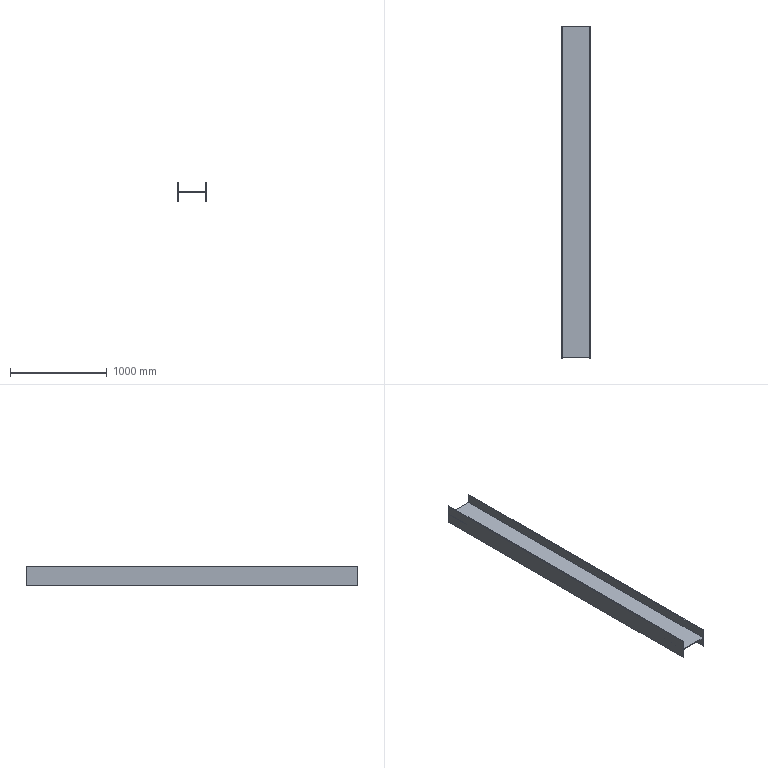Component | NX | F2 | 1 solid | 14 faces | box 300 x 3440 x 200 mm | volume 18823680 mm3 | plane 14
STEP:
#1=CARTESIAN_POINT('',(0.,0.,0.));
#2=DIRECTION('',(0.,0.,1.));
#3=DIRECTION('',(1.,0.,0.));
#4=AXIS2_PLACEMENT_3D('',#1,#2,#3);
#5=CARTESIAN_POINT('',(6772.,-266.,1440.));
#6=VERTEX_POINT('',#5);
#7=CARTESIAN_POINT('',(6772.,-266.,1536.));
#8=VERTEX_POINT('',#7);
#9=CARTESIAN_POINT('',(6772.,-266.,1440.));
#10=DIRECTION('',(0.,0.,1.));
#11=VECTOR('',#10,1.);
#12=LINE('',#9,#11);
#13=CARTESIAN_POINT('',(6772.,-3706.,1440.));
#14=DIRECTION('',(-1.,0.,0.));
#15=DIRECTION('',(0.,1.,0.));
#16=AXIS2_PLACEMENT_3D('',#13,#14,#15);
#17=PLANE('',#16);
#18=CARTESIAN_POINT('',(3440.,0.));
#19=DIRECTION('',(0.,-1.));
#20=VECTOR('',#19,1.);
#21=LINE('',#18,#20);
#22=(GEOMETRIC_REPRESENTATION_CONTEXT(2)PARAMETRIC_REPRESENTATION_CONTEXT()REPRESENTATION_CONTEXT('',''));
#23=DEFINITIONAL_REPRESENTATION('',(#21),#22);
#24=PCURVE('',#17,#23);
#25=CARTESIAN_POINT('',(6480.,-266.,1640.));
#26=DIRECTION('',(0.,-1.,0.));
#27=DIRECTION('',(-1.,0.,0.));
#28=AXIS2_PLACEMENT_3D('',#25,#26,#27);
#29=PLANE('',#28);
#30=CARTESIAN_POINT('',(-292.,200.));
#31=DIRECTION('',(0.,-1.));
#32=VECTOR('',#31,1.);
#33=LINE('',#30,#32);
#34=(GEOMETRIC_REPRESENTATION_CONTEXT(2)PARAMETRIC_REPRESENTATION_CONTEXT()REPRESENTATION_CONTEXT('',''));
#35=DEFINITIONAL_REPRESENTATION('',(#33),#34);
#36=PCURVE('',#29,#35);
#37=SURFACE_CURVE('',#12,(#24,#36),.PCURVE_S1.);
#38=EDGE_CURVE('',#6,#8,#37,.T.);
#39=ORIENTED_EDGE('',*,*,#38,.F.);
#40=CARTESIAN_POINT('',(6772.,-3706.,1440.));
#41=VERTEX_POINT('',#40);
#42=CARTESIAN_POINT('',(6772.,-3706.,1440.));
#43=DIRECTION('',(0.,1.,0.));
#44=VECTOR('',#43,1.);
#45=LINE('',#42,#44);
#46=CARTESIAN_POINT('',(0.,0.));
#47=DIRECTION('',(1.,0.));
#48=VECTOR('',#47,1.);
#49=LINE('',#46,#48);
#50=(GEOMETRIC_REPRESENTATION_CONTEXT(2)PARAMETRIC_REPRESENTATION_CONTEXT()REPRESENTATION_CONTEXT('',''));
#51=DEFINITIONAL_REPRESENTATION('',(#49),#50);
#52=PCURVE('',#17,#51);
#53=CARTESIAN_POINT('',(6780.,-3706.,1440.));
#54=DIRECTION('',(0.,0.,-1.));
#55=DIRECTION('',(0.,1.,0.));
#56=AXIS2_PLACEMENT_3D('',#53,#54,#55);
#57=PLANE('',#56);
#58=CARTESIAN_POINT('',(0.,-8.));
#59=DIRECTION('',(1.,0.));
#60=VECTOR('',#59,1.);
#61=LINE('',#58,#60);
#62=(GEOMETRIC_REPRESENTATION_CONTEXT(2)PARAMETRIC_REPRESENTATION_CONTEXT()REPRESENTATION_CONTEXT('',''));
#63=DEFINITIONAL_REPRESENTATION('',(#61),#62);
#64=PCURVE('',#57,#63);
#65=SURFACE_CURVE('',#45,(#52,#64),.PCURVE_S1.);
#66=EDGE_CURVE('',#41,#6,#65,.T.);
#67=ORIENTED_EDGE('',*,*,#66,.F.);
#68=CARTESIAN_POINT('',(6772.,-3706.,1536.));
#69=VERTEX_POINT('',#68);
#70=CARTESIAN_POINT('',(6772.,-3706.,1440.));
#71=DIRECTION('',(0.,0.,1.));
#72=VECTOR('',#71,1.);
#73=LINE('',#70,#72);
#74=CARTESIAN_POINT('',(0.,0.));
#75=DIRECTION('',(0.,-1.));
#76=VECTOR('',#75,1.);
#77=LINE('',#74,#76);
#78=(GEOMETRIC_REPRESENTATION_CONTEXT(2)PARAMETRIC_REPRESENTATION_CONTEXT()REPRESENTATION_CONTEXT('',''));
#79=DEFINITIONAL_REPRESENTATION('',(#77),#78);
#80=PCURVE('',#17,#79);
#81=CARTESIAN_POINT('',(6480.,-3706.,1640.));
#82=DIRECTION('',(0.,-1.,0.));
#83=DIRECTION('',(-1.,0.,0.));
#84=AXIS2_PLACEMENT_3D('',#81,#82,#83);
#85=PLANE('',#84);
#86=CARTESIAN_POINT('',(-292.,200.));
#87=DIRECTION('',(0.,-1.));
#88=VECTOR('',#87,1.);
#89=LINE('',#86,#88);
#90=(GEOMETRIC_REPRESENTATION_CONTEXT(2)PARAMETRIC_REPRESENTATION_CONTEXT()REPRESENTATION_CONTEXT('',''));
#91=DEFINITIONAL_REPRESENTATION('',(#89),#90);
#92=PCURVE('',#85,#91);
#93=SURFACE_CURVE('',#73,(#80,#92),.PCURVE_S1.);
#94=EDGE_CURVE('',#41,#69,#93,.T.);
#95=ORIENTED_EDGE('',*,*,#94,.T.);
#96=CARTESIAN_POINT('',(6772.,-3706.,1536.));
#97=DIRECTION('',(0.,1.,0.));
#98=VECTOR('',#97,1.);
#99=LINE('',#96,#98);
#100=CARTESIAN_POINT('',(0.,-96.));
#101=DIRECTION('',(1.,0.));
#102=VECTOR('',#101,1.);
#103=LINE('',#100,#102);
#104=(GEOMETRIC_REPRESENTATION_CONTEXT(2)PARAMETRIC_REPRESENTATION_CONTEXT()REPRESENTATION_CONTEXT('',''));
#105=DEFINITIONAL_REPRESENTATION('',(#103),#104);
#106=PCURVE('',#17,#105);
#107=CARTESIAN_POINT('',(6772.,-3706.,1536.));
#108=DIRECTION('',(0.,0.,-1.));
#109=DIRECTION('',(0.,1.,0.));
#110=AXIS2_PLACEMENT_3D('',#107,#108,#109);
#111=PLANE('',#110);
#112=CARTESIAN_POINT('',(0.,0.));
#113=DIRECTION('',(1.,0.));
#114=VECTOR('',#113,1.);
#115=LINE('',#112,#114);
#116=(GEOMETRIC_REPRESENTATION_CONTEXT(2)PARAMETRIC_REPRESENTATION_CONTEXT()REPRESENTATION_CONTEXT('',''));
#117=DEFINITIONAL_REPRESENTATION('',(#115),#116);
#118=PCURVE('',#111,#117);
#119=SURFACE_CURVE('',#99,(#106,#118),.PCURVE_S1.);
#120=EDGE_CURVE('',#69,#8,#119,.T.);
#121=ORIENTED_EDGE('',*,*,#120,.T.);
#122=EDGE_LOOP('',(#39,#67,#95,#121));
#123=FACE_BOUND('',#122,.T.);
#124=ADVANCED_FACE('',(#123),#17,.T.);
#125=CARTESIAN_POINT('',(6488.,-266.,1536.));
#126=VERTEX_POINT('',#125);
#127=CARTESIAN_POINT('',(6772.,-266.,1536.));
#128=DIRECTION('',(-1.,0.,0.));
#129=VECTOR('',#128,1.);
#130=LINE('',#127,#129);
#131=CARTESIAN_POINT('',(3440.,0.));
#132=DIRECTION('',(0.,-1.));
#133=VECTOR('',#132,1.);
#134=LINE('',#131,#133);
#135=(GEOMETRIC_REPRESENTATION_CONTEXT(2)PARAMETRIC_REPRESENTATION_CONTEXT()REPRESENTATION_CONTEXT('',''));
#136=DEFINITIONAL_REPRESENTATION('',(#134),#135);
#137=PCURVE('',#111,#136);
#138=CARTESIAN_POINT('',(-292.,104.));
#139=DIRECTION('',(1.,0.));
#140=VECTOR('',#139,1.);
#141=LINE('',#138,#140);
#142=(GEOMETRIC_REPRESENTATION_CONTEXT(2)PARAMETRIC_REPRESENTATION_CONTEXT()REPRESENTATION_CONTEXT('',''));
#143=DEFINITIONAL_REPRESENTATION('',(#141),#142);
#144=PCURVE('',#29,#143);
#145=SURFACE_CURVE('',#130,(#137,#144),.PCURVE_S1.);
#146=EDGE_CURVE('',#8,#126,#145,.T.);
#147=ORIENTED_EDGE('',*,*,#146,.F.);
#148=ORIENTED_EDGE('',*,*,#120,.F.);
#149=CARTESIAN_POINT('',(6488.,-3706.,1536.));
#150=VERTEX_POINT('',#149);
#151=CARTESIAN_POINT('',(6772.,-3706.,1536.));
#152=DIRECTION('',(-1.,0.,0.));
#153=VECTOR('',#152,1.);
#154=LINE('',#151,#153);
#155=CARTESIAN_POINT('',(0.,0.));
#156=DIRECTION('',(0.,-1.));
#157=VECTOR('',#156,1.);
#158=LINE('',#155,#157);
#159=(GEOMETRIC_REPRESENTATION_CONTEXT(2)PARAMETRIC_REPRESENTATION_CONTEXT()REPRESENTATION_CONTEXT('',''));
#160=DEFINITIONAL_REPRESENTATION('',(#158),#159);
#161=PCURVE('',#111,#160);
#162=CARTESIAN_POINT('',(-292.,104.));
#163=DIRECTION('',(1.,0.));
#164=VECTOR('',#163,1.);
#165=LINE('',#162,#164);
#166=(GEOMETRIC_REPRESENTATION_CONTEXT(2)PARAMETRIC_REPRESENTATION_CONTEXT()REPRESENTATION_CONTEXT('',''));
#167=DEFINITIONAL_REPRESENTATION('',(#165),#166);
#168=PCURVE('',#85,#167);
#169=SURFACE_CURVE('',#154,(#161,#168),.PCURVE_S1.);
#170=EDGE_CURVE('',#69,#150,#169,.T.);
#171=ORIENTED_EDGE('',*,*,#170,.T.);
#172=CARTESIAN_POINT('',(6488.,-3706.,1536.));
#173=DIRECTION('',(0.,1.,0.));
#174=VECTOR('',#173,1.);
#175=LINE('',#172,#174);
#176=CARTESIAN_POINT('',(0.,-284.));
#177=DIRECTION('',(1.,0.));
#178=VECTOR('',#177,1.);
#179=LINE('',#176,#178);
#180=(GEOMETRIC_REPRESENTATION_CONTEXT(2)PARAMETRIC_REPRESENTATION_CONTEXT()REPRESENTATION_CONTEXT('',''));
#181=DEFINITIONAL_REPRESENTATION('',(#179),#180);
#182=PCURVE('',#111,#181);
#183=CARTESIAN_POINT('',(6488.,-3706.,1536.));
#184=DIRECTION('',(1.,0.,0.));
#185=DIRECTION('',(0.,-1.,0.));
#186=AXIS2_PLACEMENT_3D('',#183,#184,#185);
#187=PLANE('',#186);
#188=CARTESIAN_POINT('',(0.,0.));
#189=DIRECTION('',(-1.,0.));
#190=VECTOR('',#189,1.);
#191=LINE('',#188,#190);
#192=(GEOMETRIC_REPRESENTATION_CONTEXT(2)PARAMETRIC_REPRESENTATION_CONTEXT()REPRESENTATION_CONTEXT('',''));
#193=DEFINITIONAL_REPRESENTATION('',(#191),#192);
#194=PCURVE('',#187,#193);
#195=SURFACE_CURVE('',#175,(#182,#194),.PCURVE_S1.);
#196=EDGE_CURVE('',#150,#126,#195,.T.);
#197=ORIENTED_EDGE('',*,*,#196,.T.);
#198=EDGE_LOOP('',(#147,#148,#171,#197));
#199=FACE_BOUND('',#198,.T.);
#200=ADVANCED_FACE('',(#199),#111,.T.);
#201=CARTESIAN_POINT('',(6488.,-266.,1440.));
#202=VERTEX_POINT('',#201);
#203=CARTESIAN_POINT('',(6488.,-266.,1536.));
#204=DIRECTION('',(0.,0.,-1.));
#205=VECTOR('',#204,1.);
#206=LINE('',#203,#205);
#207=CARTESIAN_POINT('',(-3440.,0.));
#208=DIRECTION('',(0.,1.));
#209=VECTOR('',#208,1.);
#210=LINE('',#207,#209);
#211=(GEOMETRIC_REPRESENTATION_CONTEXT(2)PARAMETRIC_REPRESENTATION_CONTEXT()REPRESENTATION_CONTEXT('',''));
#212=DEFINITIONAL_REPRESENTATION('',(#210),#211);
#213=PCURVE('',#187,#212);
#214=CARTESIAN_POINT('',(-8.,104.));
#215=DIRECTION('',(0.,1.));
#216=VECTOR('',#215,1.);
#217=LINE('',#214,#216);
#218=(GEOMETRIC_REPRESENTATION_CONTEXT(2)PARAMETRIC_REPRESENTATION_CONTEXT()REPRESENTATION_CONTEXT('',''));
#219=DEFINITIONAL_REPRESENTATION('',(#217),#218);
#220=PCURVE('',#29,#219);
#221=SURFACE_CURVE('',#206,(#213,#220),.PCURVE_S1.);
#222=EDGE_CURVE('',#126,#202,#221,.T.);
#223=ORIENTED_EDGE('',*,*,#222,.F.);
#224=ORIENTED_EDGE('',*,*,#196,.F.);
#225=CARTESIAN_POINT('',(6488.,-3706.,1440.));
#226=VERTEX_POINT('',#225);
#227=CARTESIAN_POINT('',(6488.,-3706.,1536.));
#228=DIRECTION('',(0.,0.,-1.));
#229=VECTOR('',#228,1.);
#230=LINE('',#227,#229);
#231=CARTESIAN_POINT('',(0.,0.));
#232=DIRECTION('',(0.,1.));
#233=VECTOR('',#232,1.);
#234=LINE('',#231,#233);
#235=(GEOMETRIC_REPRESENTATION_CONTEXT(2)PARAMETRIC_REPRESENTATION_CONTEXT()REPRESENTATION_CONTEXT('',''));
#236=DEFINITIONAL_REPRESENTATION('',(#234),#235);
#237=PCURVE('',#187,#236);
#238=CARTESIAN_POINT('',(-8.,104.));
#239=DIRECTION('',(0.,1.));
#240=VECTOR('',#239,1.);
#241=LINE('',#238,#240);
#242=(GEOMETRIC_REPRESENTATION_CONTEXT(2)PARAMETRIC_REPRESENTATION_CONTEXT()REPRESENTATION_CONTEXT('',''));
#243=DEFINITIONAL_REPRESENTATION('',(#241),#242);
#244=PCURVE('',#85,#243);
#245=SURFACE_CURVE('',#230,(#237,#244),.PCURVE_S1.);
#246=EDGE_CURVE('',#150,#226,#245,.T.);
#247=ORIENTED_EDGE('',*,*,#246,.T.);
#248=CARTESIAN_POINT('',(6488.,-3706.,1440.));
#249=DIRECTION('',(0.,1.,0.));
#250=VECTOR('',#249,1.);
#251=LINE('',#248,#250);
#252=CARTESIAN_POINT('',(0.,96.));
#253=DIRECTION('',(-1.,0.));
#254=VECTOR('',#253,1.);
#255=LINE('',#252,#254);
#256=(GEOMETRIC_REPRESENTATION_CONTEXT(2)PARAMETRIC_REPRESENTATION_CONTEXT()REPRESENTATION_CONTEXT('',''));
#257=DEFINITIONAL_REPRESENTATION('',(#255),#256);
#258=PCURVE('',#187,#257);
#259=CARTESIAN_POINT('',(6488.,-3706.,1440.));
#260=DIRECTION('',(0.,0.,-1.));
#261=DIRECTION('',(0.,1.,0.));
#262=AXIS2_PLACEMENT_3D('',#259,#260,#261);
#263=PLANE('',#262);
#264=CARTESIAN_POINT('',(0.,0.));
#265=DIRECTION('',(1.,0.));
#266=VECTOR('',#265,1.);
#267=LINE('',#264,#266);
#268=(GEOMETRIC_REPRESENTATION_CONTEXT(2)PARAMETRIC_REPRESENTATION_CONTEXT()REPRESENTATION_CONTEXT('',''));
#269=DEFINITIONAL_REPRESENTATION('',(#267),#268);
#270=PCURVE('',#263,#269);
#271=SURFACE_CURVE('',#251,(#258,#270),.PCURVE_S1.);
#272=EDGE_CURVE('',#226,#202,#271,.T.);
#273=ORIENTED_EDGE('',*,*,#272,.T.);
#274=EDGE_LOOP('',(#223,#224,#247,#273));
#275=FACE_BOUND('',#274,.T.);
#276=ADVANCED_FACE('',(#275),#187,.T.);
#277=CARTESIAN_POINT('',(6480.,-266.,1440.));
#278=VERTEX_POINT('',#277);
#279=CARTESIAN_POINT('',(6488.,-266.,1440.));
#280=DIRECTION('',(-1.,0.,0.));
#281=VECTOR('',#280,1.);
#282=LINE('',#279,#281);
#283=CARTESIAN_POINT('',(3440.,0.));
#284=DIRECTION('',(0.,-1.));
#285=VECTOR('',#284,1.);
#286=LINE('',#283,#285);
#287=(GEOMETRIC_REPRESENTATION_CONTEXT(2)PARAMETRIC_REPRESENTATION_CONTEXT()REPRESENTATION_CONTEXT('',''));
#288=DEFINITIONAL_REPRESENTATION('',(#286),#287);
#289=PCURVE('',#263,#288);
#290=CARTESIAN_POINT('',(-8.,200.));
#291=DIRECTION('',(1.,0.));
#292=VECTOR('',#291,1.);
#293=LINE('',#290,#292);
#294=(GEOMETRIC_REPRESENTATION_CONTEXT(2)PARAMETRIC_REPRESENTATION_CONTEXT()REPRESENTATION_CONTEXT('',''));
#295=DEFINITIONAL_REPRESENTATION('',(#293),#294);
#296=PCURVE('',#29,#295);
#297=SURFACE_CURVE('',#282,(#289,#296),.PCURVE_S1.);
#298=EDGE_CURVE('',#202,#278,#297,.T.);
#299=ORIENTED_EDGE('',*,*,#298,.F.);
#300=ORIENTED_EDGE('',*,*,#272,.F.);
#301=CARTESIAN_POINT('',(6480.,-3706.,1440.));
#302=VERTEX_POINT('',#301);
#303=CARTESIAN_POINT('',(6488.,-3706.,1440.));
#304=DIRECTION('',(-1.,0.,0.));
#305=VECTOR('',#304,1.);
#306=LINE('',#303,#305);
#307=CARTESIAN_POINT('',(0.,0.));
#308=DIRECTION('',(0.,-1.));
#309=VECTOR('',#308,1.);
#310=LINE('',#307,#309);
#311=(GEOMETRIC_REPRESENTATION_CONTEXT(2)PARAMETRIC_REPRESENTATION_CONTEXT()REPRESENTATION_CONTEXT('',''));
#312=DEFINITIONAL_REPRESENTATION('',(#310),#311);
#313=PCURVE('',#263,#312);
#314=CARTESIAN_POINT('',(-8.,200.));
#315=DIRECTION('',(1.,0.));
#316=VECTOR('',#315,1.);
#317=LINE('',#314,#316);
#318=(GEOMETRIC_REPRESENTATION_CONTEXT(2)PARAMETRIC_REPRESENTATION_CONTEXT()REPRESENTATION_CONTEXT('',''));
#319=DEFINITIONAL_REPRESENTATION('',(#317),#318);
#320=PCURVE('',#85,#319);
#321=SURFACE_CURVE('',#306,(#313,#320),.PCURVE_S1.);
#322=EDGE_CURVE('',#226,#302,#321,.T.);
#323=ORIENTED_EDGE('',*,*,#322,.T.);
#324=CARTESIAN_POINT('',(6480.,-3706.,1440.));
#325=DIRECTION('',(0.,1.,0.));
#326=VECTOR('',#325,1.);
#327=LINE('',#324,#326);
#328=CARTESIAN_POINT('',(0.,-8.));
#329=DIRECTION('',(1.,0.));
#330=VECTOR('',#329,1.);
#331=LINE('',#328,#330);
#332=(GEOMETRIC_REPRESENTATION_CONTEXT(2)PARAMETRIC_REPRESENTATION_CONTEXT()REPRESENTATION_CONTEXT('',''));
#333=DEFINITIONAL_REPRESENTATION('',(#331),#332);
#334=PCURVE('',#263,#333);
#335=CARTESIAN_POINT('',(6480.,-3706.,1440.));
#336=DIRECTION('',(-1.,0.,0.));
#337=DIRECTION('',(0.,1.,0.));
#338=AXIS2_PLACEMENT_3D('',#335,#336,#337);
#339=PLANE('',#338);
#340=CARTESIAN_POINT('',(0.,0.));
#341=DIRECTION('',(1.,0.));
#342=VECTOR('',#341,1.);
#343=LINE('',#340,#342);
#344=(GEOMETRIC_REPRESENTATION_CONTEXT(2)PARAMETRIC_REPRESENTATION_CONTEXT()REPRESENTATION_CONTEXT('',''));
#345=DEFINITIONAL_REPRESENTATION('',(#343),#344);
#346=PCURVE('',#339,#345);
#347=SURFACE_CURVE('',#327,(#334,#346),.PCURVE_S1.);
#348=EDGE_CURVE('',#302,#278,#347,.T.);
#349=ORIENTED_EDGE('',*,*,#348,.T.);
#350=EDGE_LOOP('',(#299,#300,#323,#349));
#351=FACE_BOUND('',#350,.T.);
#352=ADVANCED_FACE('',(#351),#263,.T.);
#353=CARTESIAN_POINT('',(6480.,-266.,1640.));
#354=VERTEX_POINT('',#353);
#355=CARTESIAN_POINT('',(6480.,-266.,1440.));
#356=DIRECTION('',(0.,0.,1.));
#357=VECTOR('',#356,1.);
#358=LINE('',#355,#357);
#359=CARTESIAN_POINT('',(3440.,0.));
#360=DIRECTION('',(0.,-1.));
#361=VECTOR('',#360,1.);
#362=LINE('',#359,#361);
#363=(GEOMETRIC_REPRESENTATION_CONTEXT(2)PARAMETRIC_REPRESENTATION_CONTEXT()REPRESENTATION_CONTEXT('',''));
#364=DEFINITIONAL_REPRESENTATION('',(#362),#363);
#365=PCURVE('',#339,#364);
#366=CARTESIAN_POINT('',(0.,200.));
#367=DIRECTION('',(0.,-1.));
#368=VECTOR('',#367,1.);
#369=LINE('',#366,#368);
#370=(GEOMETRIC_REPRESENTATION_CONTEXT(2)PARAMETRIC_REPRESENTATION_CONTEXT()REPRESENTATION_CONTEXT('',''));
#371=DEFINITIONAL_REPRESENTATION('',(#369),#370);
#372=PCURVE('',#29,#371);
#373=SURFACE_CURVE('',#358,(#365,#372),.PCURVE_S1.);
#374=EDGE_CURVE('',#278,#354,#373,.T.);
#375=ORIENTED_EDGE('',*,*,#374,.F.);
#376=ORIENTED_EDGE('',*,*,#348,.F.);
#377=CARTESIAN_POINT('',(6480.,-3706.,1640.));
#378=VERTEX_POINT('',#377);
#379=CARTESIAN_POINT('',(6480.,-3706.,1440.));
#380=DIRECTION('',(0.,0.,1.));
#381=VECTOR('',#380,1.);
#382=LINE('',#379,#381);
#383=CARTESIAN_POINT('',(0.,0.));
#384=DIRECTION('',(0.,-1.));
#385=VECTOR('',#384,1.);
#386=LINE('',#383,#385);
#387=(GEOMETRIC_REPRESENTATION_CONTEXT(2)PARAMETRIC_REPRESENTATION_CONTEXT()REPRESENTATION_CONTEXT('',''));
#388=DEFINITIONAL_REPRESENTATION('',(#386),#387);
#389=PCURVE('',#339,#388);
#390=CARTESIAN_POINT('',(0.,200.));
#391=DIRECTION('',(0.,-1.));
#392=VECTOR('',#391,1.);
#393=LINE('',#390,#392);
#394=(GEOMETRIC_REPRESENTATION_CONTEXT(2)PARAMETRIC_REPRESENTATION_CONTEXT()REPRESENTATION_CONTEXT('',''));
#395=DEFINITIONAL_REPRESENTATION('',(#393),#394);
#396=PCURVE('',#85,#395);
#397=SURFACE_CURVE('',#382,(#389,#396),.PCURVE_S1.);
#398=EDGE_CURVE('',#302,#378,#397,.T.);
#399=ORIENTED_EDGE('',*,*,#398,.T.);
#400=CARTESIAN_POINT('',(6480.,-3706.,1640.));
#401=DIRECTION('',(0.,1.,0.));
#402=VECTOR('',#401,1.);
#403=LINE('',#400,#402);
#404=CARTESIAN_POINT('',(0.,-200.));
#405=DIRECTION('',(1.,0.));
#406=VECTOR('',#405,1.);
#407=LINE('',#404,#406);
#408=(GEOMETRIC_REPRESENTATION_CONTEXT(2)PARAMETRIC_REPRESENTATION_CONTEXT()REPRESENTATION_CONTEXT('',''));
#409=DEFINITIONAL_REPRESENTATION('',(#407),#408);
#410=PCURVE('',#339,#409);
#411=CARTESIAN_POINT('',(6480.,-3706.,1640.));
#412=DIRECTION('',(0.,0.,1.));
#413=DIRECTION('',(0.,-1.,0.));
#414=AXIS2_PLACEMENT_3D('',#411,#412,#413);
#415=PLANE('',#414);
#416=CARTESIAN_POINT('',(0.,0.));
#417=DIRECTION('',(-1.,0.));
#418=VECTOR('',#417,1.);
#419=LINE('',#416,#418);
#420=(GEOMETRIC_REPRESENTATION_CONTEXT(2)PARAMETRIC_REPRESENTATION_CONTEXT()REPRESENTATION_CONTEXT('',''));
#421=DEFINITIONAL_REPRESENTATION('',(#419),#420);
#422=PCURVE('',#415,#421);
#423=SURFACE_CURVE('',#403,(#410,#422),.PCURVE_S1.);
#424=EDGE_CURVE('',#378,#354,#423,.T.);
#425=ORIENTED_EDGE('',*,*,#424,.T.);
#426=EDGE_LOOP('',(#375,#376,#399,#425));
#427=FACE_BOUND('',#426,.T.);
#428=ADVANCED_FACE('',(#427),#339,.T.);
#429=CARTESIAN_POINT('',(6488.,-266.,1640.));
#430=VERTEX_POINT('',#429);
#431=CARTESIAN_POINT('',(6480.,-266.,1640.));
#432=DIRECTION('',(1.,0.,0.));
#433=VECTOR('',#432,1.);
#434=LINE('',#431,#433);
#435=CARTESIAN_POINT('',(-3440.,0.));
#436=DIRECTION('',(0.,1.));
#437=VECTOR('',#436,1.);
#438=LINE('',#435,#437);
#439=(GEOMETRIC_REPRESENTATION_CONTEXT(2)PARAMETRIC_REPRESENTATION_CONTEXT()REPRESENTATION_CONTEXT('',''));
#440=DEFINITIONAL_REPRESENTATION('',(#438),#439);
#441=PCURVE('',#415,#440);
#442=CARTESIAN_POINT('',(0.,0.));
#443=DIRECTION('',(-1.,0.));
#444=VECTOR('',#443,1.);
#445=LINE('',#442,#444);
#446=(GEOMETRIC_REPRESENTATION_CONTEXT(2)PARAMETRIC_REPRESENTATION_CONTEXT()REPRESENTATION_CONTEXT('',''));
#447=DEFINITIONAL_REPRESENTATION('',(#445),#446);
#448=PCURVE('',#29,#447);
#449=SURFACE_CURVE('',#434,(#441,#448),.PCURVE_S1.);
#450=EDGE_CURVE('',#354,#430,#449,.T.);
#451=ORIENTED_EDGE('',*,*,#450,.F.);
#452=ORIENTED_EDGE('',*,*,#424,.F.);
#453=CARTESIAN_POINT('',(6488.,-3706.,1640.));
#454=VERTEX_POINT('',#453);
#455=CARTESIAN_POINT('',(6480.,-3706.,1640.));
#456=DIRECTION('',(1.,0.,0.));
#457=VECTOR('',#456,1.);
#458=LINE('',#455,#457);
#459=CARTESIAN_POINT('',(0.,0.));
#460=DIRECTION('',(0.,1.));
#461=VECTOR('',#460,1.);
#462=LINE('',#459,#461);
#463=(GEOMETRIC_REPRESENTATION_CONTEXT(2)PARAMETRIC_REPRESENTATION_CONTEXT()REPRESENTATION_CONTEXT('',''));
#464=DEFINITIONAL_REPRESENTATION('',(#462),#463);
#465=PCURVE('',#415,#464);
#466=CARTESIAN_POINT('',(0.,0.));
#467=DIRECTION('',(-1.,0.));
#468=VECTOR('',#467,1.);
#469=LINE('',#466,#468);
#470=(GEOMETRIC_REPRESENTATION_CONTEXT(2)PARAMETRIC_REPRESENTATION_CONTEXT()REPRESENTATION_CONTEXT('',''));
#471=DEFINITIONAL_REPRESENTATION('',(#469),#470);
#472=PCURVE('',#85,#471);
#473=SURFACE_CURVE('',#458,(#465,#472),.PCURVE_S1.);
#474=EDGE_CURVE('',#378,#454,#473,.T.);
#475=ORIENTED_EDGE('',*,*,#474,.T.);
#476=CARTESIAN_POINT('',(6488.,-3706.,1640.));
#477=DIRECTION('',(0.,1.,0.));
#478=VECTOR('',#477,1.);
#479=LINE('',#476,#478);
#480=CARTESIAN_POINT('',(0.,8.));
#481=DIRECTION('',(-1.,0.));
#482=VECTOR('',#481,1.);
#483=LINE('',#480,#482);
#484=(GEOMETRIC_REPRESENTATION_CONTEXT(2)PARAMETRIC_REPRESENTATION_CONTEXT()REPRESENTATION_CONTEXT('',''));
#485=DEFINITIONAL_REPRESENTATION('',(#483),#484);
#486=PCURVE('',#415,#485);
#487=CARTESIAN_POINT('',(6488.,-3706.,1640.));
#488=DIRECTION('',(1.,0.,0.));
#489=DIRECTION('',(0.,-1.,0.));
#490=AXIS2_PLACEMENT_3D('',#487,#488,#489);
#491=PLANE('',#490);
#492=CARTESIAN_POINT('',(0.,0.));
#493=DIRECTION('',(-1.,0.));
#494=VECTOR('',#493,1.);
#495=LINE('',#492,#494);
#496=(GEOMETRIC_REPRESENTATION_CONTEXT(2)PARAMETRIC_REPRESENTATION_CONTEXT()REPRESENTATION_CONTEXT('',''));
#497=DEFINITIONAL_REPRESENTATION('',(#495),#496);
#498=PCURVE('',#491,#497);
#499=SURFACE_CURVE('',#479,(#486,#498),.PCURVE_S1.);
#500=EDGE_CURVE('',#454,#430,#499,.T.);
#501=ORIENTED_EDGE('',*,*,#500,.T.);
#502=EDGE_LOOP('',(#451,#452,#475,#501));
#503=FACE_BOUND('',#502,.T.);
#504=ADVANCED_FACE('',(#503),#415,.T.);
#505=CARTESIAN_POINT('',(6488.,-266.,1544.));
#506=VERTEX_POINT('',#505);
#507=CARTESIAN_POINT('',(6488.,-266.,1640.));
#508=DIRECTION('',(0.,0.,-1.));
#509=VECTOR('',#508,1.);
#510=LINE('',#507,#509);
#511=CARTESIAN_POINT('',(-3440.,0.));
#512=DIRECTION('',(0.,1.));
#513=VECTOR('',#512,1.);
#514=LINE('',#511,#513);
#515=(GEOMETRIC_REPRESENTATION_CONTEXT(2)PARAMETRIC_REPRESENTATION_CONTEXT()REPRESENTATION_CONTEXT('',''));
#516=DEFINITIONAL_REPRESENTATION('',(#514),#515);
#517=PCURVE('',#491,#516);
#518=CARTESIAN_POINT('',(-8.,0.));
#519=DIRECTION('',(0.,1.));
#520=VECTOR('',#519,1.);
#521=LINE('',#518,#520);
#522=(GEOMETRIC_REPRESENTATION_CONTEXT(2)PARAMETRIC_REPRESENTATION_CONTEXT()REPRESENTATION_CONTEXT('',''));
#523=DEFINITIONAL_REPRESENTATION('',(#521),#522);
#524=PCURVE('',#29,#523);
#525=SURFACE_CURVE('',#510,(#517,#524),.PCURVE_S1.);
#526=EDGE_CURVE('',#430,#506,#525,.T.);
#527=ORIENTED_EDGE('',*,*,#526,.F.);
#528=ORIENTED_EDGE('',*,*,#500,.F.);
#529=CARTESIAN_POINT('',(6488.,-3706.,1544.));
#530=VERTEX_POINT('',#529);
#531=CARTESIAN_POINT('',(6488.,-3706.,1640.));
#532=DIRECTION('',(0.,0.,-1.));
#533=VECTOR('',#532,1.);
#534=LINE('',#531,#533);
#535=CARTESIAN_POINT('',(0.,0.));
#536=DIRECTION('',(0.,1.));
#537=VECTOR('',#536,1.);
#538=LINE('',#535,#537);
#539=(GEOMETRIC_REPRESENTATION_CONTEXT(2)PARAMETRIC_REPRESENTATION_CONTEXT()REPRESENTATION_CONTEXT('',''));
#540=DEFINITIONAL_REPRESENTATION('',(#538),#539);
#541=PCURVE('',#491,#540);
#542=CARTESIAN_POINT('',(-8.,0.));
#543=DIRECTION('',(0.,1.));
#544=VECTOR('',#543,1.);
#545=LINE('',#542,#544);
#546=(GEOMETRIC_REPRESENTATION_CONTEXT(2)PARAMETRIC_REPRESENTATION_CONTEXT()REPRESENTATION_CONTEXT('',''));
#547=DEFINITIONAL_REPRESENTATION('',(#545),#546);
#548=PCURVE('',#85,#547);
#549=SURFACE_CURVE('',#534,(#541,#548),.PCURVE_S1.);
#550=EDGE_CURVE('',#454,#530,#549,.T.);
#551=ORIENTED_EDGE('',*,*,#550,.T.);
#552=CARTESIAN_POINT('',(6488.,-3706.,1544.));
#553=DIRECTION('',(0.,1.,0.));
#554=VECTOR('',#553,1.);
#555=LINE('',#552,#554);
#556=CARTESIAN_POINT('',(0.,96.));
#557=DIRECTION('',(-1.,0.));
#558=VECTOR('',#557,1.);
#559=LINE('',#556,#558);
#560=(GEOMETRIC_REPRESENTATION_CONTEXT(2)PARAMETRIC_REPRESENTATION_CONTEXT()REPRESENTATION_CONTEXT('',''));
#561=DEFINITIONAL_REPRESENTATION('',(#559),#560);
#562=PCURVE('',#491,#561);
#563=CARTESIAN_POINT('',(6488.,-3706.,1544.));
#564=DIRECTION('',(0.,0.,1.));
#565=DIRECTION('',(0.,-1.,0.));
#566=AXIS2_PLACEMENT_3D('',#563,#564,#565);
#567=PLANE('',#566);
#568=CARTESIAN_POINT('',(0.,0.));
#569=DIRECTION('',(-1.,0.));
#570=VECTOR('',#569,1.);
#571=LINE('',#568,#570);
#572=(GEOMETRIC_REPRESENTATION_CONTEXT(2)PARAMETRIC_REPRESENTATION_CONTEXT()REPRESENTATION_CONTEXT('',''));
#573=DEFINITIONAL_REPRESENTATION('',(#571),#572);
#574=PCURVE('',#567,#573);
#575=SURFACE_CURVE('',#555,(#562,#574),.PCURVE_S1.);
#576=EDGE_CURVE('',#530,#506,#575,.T.);
#577=ORIENTED_EDGE('',*,*,#576,.T.);
#578=EDGE_LOOP('',(#527,#528,#551,#577));
#579=FACE_BOUND('',#578,.T.);
#580=ADVANCED_FACE('',(#579),#491,.T.);
#581=CARTESIAN_POINT('',(6772.,-266.,1544.));
#582=VERTEX_POINT('',#581);
#583=CARTESIAN_POINT('',(6488.,-266.,1544.));
#584=DIRECTION('',(1.,0.,0.));
#585=VECTOR('',#584,1.);
#586=LINE('',#583,#585);
#587=CARTESIAN_POINT('',(-3440.,0.));
#588=DIRECTION('',(0.,1.));
#589=VECTOR('',#588,1.);
#590=LINE('',#587,#589);
#591=(GEOMETRIC_REPRESENTATION_CONTEXT(2)PARAMETRIC_REPRESENTATION_CONTEXT()REPRESENTATION_CONTEXT('',''));
#592=DEFINITIONAL_REPRESENTATION('',(#590),#591);
#593=PCURVE('',#567,#592);
#594=CARTESIAN_POINT('',(-8.,96.));
#595=DIRECTION('',(-1.,0.));
#596=VECTOR('',#595,1.);
#597=LINE('',#594,#596);
#598=(GEOMETRIC_REPRESENTATION_CONTEXT(2)PARAMETRIC_REPRESENTATION_CONTEXT()REPRESENTATION_CONTEXT('',''));
#599=DEFINITIONAL_REPRESENTATION('',(#597),#598);
#600=PCURVE('',#29,#599);
#601=SURFACE_CURVE('',#586,(#593,#600),.PCURVE_S1.);
#602=EDGE_CURVE('',#506,#582,#601,.T.);
#603=ORIENTED_EDGE('',*,*,#602,.F.);
#604=ORIENTED_EDGE('',*,*,#576,.F.);
#605=CARTESIAN_POINT('',(6772.,-3706.,1544.));
#606=VERTEX_POINT('',#605);
#607=CARTESIAN_POINT('',(6488.,-3706.,1544.));
#608=DIRECTION('',(1.,0.,0.));
#609=VECTOR('',#608,1.);
#610=LINE('',#607,#609);
#611=CARTESIAN_POINT('',(0.,0.));
#612=DIRECTION('',(0.,1.));
#613=VECTOR('',#612,1.);
#614=LINE('',#611,#613);
#615=(GEOMETRIC_REPRESENTATION_CONTEXT(2)PARAMETRIC_REPRESENTATION_CONTEXT()REPRESENTATION_CONTEXT('',''));
#616=DEFINITIONAL_REPRESENTATION('',(#614),#615);
#617=PCURVE('',#567,#616);
#618=CARTESIAN_POINT('',(-8.,96.));
#619=DIRECTION('',(-1.,0.));
#620=VECTOR('',#619,1.);
#621=LINE('',#618,#620);
#622=(GEOMETRIC_REPRESENTATION_CONTEXT(2)PARAMETRIC_REPRESENTATION_CONTEXT()REPRESENTATION_CONTEXT('',''));
#623=DEFINITIONAL_REPRESENTATION('',(#621),#622);
#624=PCURVE('',#85,#623);
#625=SURFACE_CURVE('',#610,(#617,#624),.PCURVE_S1.);
#626=EDGE_CURVE('',#530,#606,#625,.T.);
#627=ORIENTED_EDGE('',*,*,#626,.T.);
#628=CARTESIAN_POINT('',(6772.,-3706.,1544.));
#629=DIRECTION('',(0.,1.,0.));
#630=VECTOR('',#629,1.);
#631=LINE('',#628,#630);
#632=CARTESIAN_POINT('',(0.,284.));
#633=DIRECTION('',(-1.,0.));
#634=VECTOR('',#633,1.);
#635=LINE('',#632,#634);
#636=(GEOMETRIC_REPRESENTATION_CONTEXT(2)PARAMETRIC_REPRESENTATION_CONTEXT()REPRESENTATION_CONTEXT('',''));
#637=DEFINITIONAL_REPRESENTATION('',(#635),#636);
#638=PCURVE('',#567,#637);
#639=CARTESIAN_POINT('',(6772.,-3706.,1544.));
#640=DIRECTION('',(-1.,0.,0.));
#641=DIRECTION('',(0.,1.,0.));
#642=AXIS2_PLACEMENT_3D('',#639,#640,#641);
#643=PLANE('',#642);
#644=CARTESIAN_POINT('',(0.,0.));
#645=DIRECTION('',(1.,0.));
#646=VECTOR('',#645,1.);
#647=LINE('',#644,#646);
#648=(GEOMETRIC_REPRESENTATION_CONTEXT(2)PARAMETRIC_REPRESENTATION_CONTEXT()REPRESENTATION_CONTEXT('',''));
#649=DEFINITIONAL_REPRESENTATION('',(#647),#648);
#650=PCURVE('',#643,#649);
#651=SURFACE_CURVE('',#631,(#638,#650),.PCURVE_S1.);
#652=EDGE_CURVE('',#606,#582,#651,.T.);
#653=ORIENTED_EDGE('',*,*,#652,.T.);
#654=EDGE_LOOP('',(#603,#604,#627,#653));
#655=FACE_BOUND('',#654,.T.);
#656=ADVANCED_FACE('',(#655),#567,.T.);
#657=CARTESIAN_POINT('',(6772.,-266.,1640.));
#658=VERTEX_POINT('',#657);
#659=CARTESIAN_POINT('',(6772.,-266.,1544.));
#660=DIRECTION('',(0.,0.,1.));
#661=VECTOR('',#660,1.);
#662=LINE('',#659,#661);
#663=CARTESIAN_POINT('',(3440.,0.));
#664=DIRECTION('',(0.,-1.));
#665=VECTOR('',#664,1.);
#666=LINE('',#663,#665);
#667=(GEOMETRIC_REPRESENTATION_CONTEXT(2)PARAMETRIC_REPRESENTATION_CONTEXT()REPRESENTATION_CONTEXT('',''));
#668=DEFINITIONAL_REPRESENTATION('',(#666),#667);
#669=PCURVE('',#643,#668);
#670=CARTESIAN_POINT('',(-292.,96.));
#671=DIRECTION('',(0.,-1.));
#672=VECTOR('',#671,1.);
#673=LINE('',#670,#672);
#674=(GEOMETRIC_REPRESENTATION_CONTEXT(2)PARAMETRIC_REPRESENTATION_CONTEXT()REPRESENTATION_CONTEXT('',''));
#675=DEFINITIONAL_REPRESENTATION('',(#673),#674);
#676=PCURVE('',#29,#675);
#677=SURFACE_CURVE('',#662,(#669,#676),.PCURVE_S1.);
#678=EDGE_CURVE('',#582,#658,#677,.T.);
#679=ORIENTED_EDGE('',*,*,#678,.F.);
#680=ORIENTED_EDGE('',*,*,#652,.F.);
#681=CARTESIAN_POINT('',(6772.,-3706.,1640.));
#682=VERTEX_POINT('',#681);
#683=CARTESIAN_POINT('',(6772.,-3706.,1544.));
#684=DIRECTION('',(0.,0.,1.));
#685=VECTOR('',#684,1.);
#686=LINE('',#683,#685);
#687=CARTESIAN_POINT('',(0.,0.));
#688=DIRECTION('',(0.,-1.));
#689=VECTOR('',#688,1.);
#690=LINE('',#687,#689);
#691=(GEOMETRIC_REPRESENTATION_CONTEXT(2)PARAMETRIC_REPRESENTATION_CONTEXT()REPRESENTATION_CONTEXT('',''));
#692=DEFINITIONAL_REPRESENTATION('',(#690),#691);
#693=PCURVE('',#643,#692);
#694=CARTESIAN_POINT('',(-292.,96.));
#695=DIRECTION('',(0.,-1.));
#696=VECTOR('',#695,1.);
#697=LINE('',#694,#696);
#698=(GEOMETRIC_REPRESENTATION_CONTEXT(2)PARAMETRIC_REPRESENTATION_CONTEXT()REPRESENTATION_CONTEXT('',''));
#699=DEFINITIONAL_REPRESENTATION('',(#697),#698);
#700=PCURVE('',#85,#699);
#701=SURFACE_CURVE('',#686,(#693,#700),.PCURVE_S1.);
#702=EDGE_CURVE('',#606,#682,#701,.T.);
#703=ORIENTED_EDGE('',*,*,#702,.T.);
#704=CARTESIAN_POINT('',(6772.,-3706.,1640.));
#705=DIRECTION('',(0.,1.,0.));
#706=VECTOR('',#705,1.);
#707=LINE('',#704,#706);
#708=CARTESIAN_POINT('',(0.,-96.));
#709=DIRECTION('',(1.,0.));
#710=VECTOR('',#709,1.);
#711=LINE('',#708,#710);
#712=(GEOMETRIC_REPRESENTATION_CONTEXT(2)PARAMETRIC_REPRESENTATION_CONTEXT()REPRESENTATION_CONTEXT('',''));
#713=DEFINITIONAL_REPRESENTATION('',(#711),#712);
#714=PCURVE('',#643,#713);
#715=CARTESIAN_POINT('',(6772.,-3706.,1640.));
#716=DIRECTION('',(0.,0.,1.));
#717=DIRECTION('',(0.,-1.,0.));
#718=AXIS2_PLACEMENT_3D('',#715,#716,#717);
#719=PLANE('',#718);
#720=CARTESIAN_POINT('',(0.,0.));
#721=DIRECTION('',(-1.,0.));
#722=VECTOR('',#721,1.);
#723=LINE('',#720,#722);
#724=(GEOMETRIC_REPRESENTATION_CONTEXT(2)PARAMETRIC_REPRESENTATION_CONTEXT()REPRESENTATION_CONTEXT('',''));
#725=DEFINITIONAL_REPRESENTATION('',(#723),#724);
#726=PCURVE('',#719,#725);
#727=SURFACE_CURVE('',#707,(#714,#726),.PCURVE_S1.);
#728=EDGE_CURVE('',#682,#658,#727,.T.);
#729=ORIENTED_EDGE('',*,*,#728,.T.);
#730=EDGE_LOOP('',(#679,#680,#703,#729));
#731=FACE_BOUND('',#730,.T.);
#732=ADVANCED_FACE('',(#731),#643,.T.);
#733=CARTESIAN_POINT('',(6780.,-266.,1640.));
#734=VERTEX_POINT('',#733);
#735=CARTESIAN_POINT('',(6772.,-266.,1640.));
#736=DIRECTION('',(1.,0.,0.));
#737=VECTOR('',#736,1.);
#738=LINE('',#735,#737);
#739=CARTESIAN_POINT('',(-3440.,0.));
#740=DIRECTION('',(0.,1.));
#741=VECTOR('',#740,1.);
#742=LINE('',#739,#741);
#743=(GEOMETRIC_REPRESENTATION_CONTEXT(2)PARAMETRIC_REPRESENTATION_CONTEXT()REPRESENTATION_CONTEXT('',''));
#744=DEFINITIONAL_REPRESENTATION('',(#742),#743);
#745=PCURVE('',#719,#744);
#746=CARTESIAN_POINT('',(-292.,0.));
#747=DIRECTION('',(-1.,0.));
#748=VECTOR('',#747,1.);
#749=LINE('',#746,#748);
#750=(GEOMETRIC_REPRESENTATION_CONTEXT(2)PARAMETRIC_REPRESENTATION_CONTEXT()REPRESENTATION_CONTEXT('',''));
#751=DEFINITIONAL_REPRESENTATION('',(#749),#750);
#752=PCURVE('',#29,#751);
#753=SURFACE_CURVE('',#738,(#745,#752),.PCURVE_S1.);
#754=EDGE_CURVE('',#658,#734,#753,.T.);
#755=ORIENTED_EDGE('',*,*,#754,.F.);
#756=ORIENTED_EDGE('',*,*,#728,.F.);
#757=CARTESIAN_POINT('',(6780.,-3706.,1640.));
#758=VERTEX_POINT('',#757);
#759=CARTESIAN_POINT('',(6772.,-3706.,1640.));
#760=DIRECTION('',(1.,0.,0.));
#761=VECTOR('',#760,1.);
#762=LINE('',#759,#761);
#763=CARTESIAN_POINT('',(0.,0.));
#764=DIRECTION('',(0.,1.));
#765=VECTOR('',#764,1.);
#766=LINE('',#763,#765);
#767=(GEOMETRIC_REPRESENTATION_CONTEXT(2)PARAMETRIC_REPRESENTATION_CONTEXT()REPRESENTATION_CONTEXT('',''));
#768=DEFINITIONAL_REPRESENTATION('',(#766),#767);
#769=PCURVE('',#719,#768);
#770=CARTESIAN_POINT('',(-292.,0.));
#771=DIRECTION('',(-1.,0.));
#772=VECTOR('',#771,1.);
#773=LINE('',#770,#772);
#774=(GEOMETRIC_REPRESENTATION_CONTEXT(2)PARAMETRIC_REPRESENTATION_CONTEXT()REPRESENTATION_CONTEXT('',''));
#775=DEFINITIONAL_REPRESENTATION('',(#773),#774);
#776=PCURVE('',#85,#775);
#777=SURFACE_CURVE('',#762,(#769,#776),.PCURVE_S1.);
#778=EDGE_CURVE('',#682,#758,#777,.T.);
#779=ORIENTED_EDGE('',*,*,#778,.T.);
#780=CARTESIAN_POINT('',(6780.,-3706.,1640.));
#781=DIRECTION('',(0.,1.,0.));
#782=VECTOR('',#781,1.);
#783=LINE('',#780,#782);
#784=CARTESIAN_POINT('',(0.,8.));
#785=DIRECTION('',(-1.,0.));
#786=VECTOR('',#785,1.);
#787=LINE('',#784,#786);
#788=(GEOMETRIC_REPRESENTATION_CONTEXT(2)PARAMETRIC_REPRESENTATION_CONTEXT()REPRESENTATION_CONTEXT('',''));
#789=DEFINITIONAL_REPRESENTATION('',(#787),#788);
#790=PCURVE('',#719,#789);
#791=CARTESIAN_POINT('',(6780.,-3706.,1640.));
#792=DIRECTION('',(1.,0.,0.));
#793=DIRECTION('',(0.,-1.,0.));
#794=AXIS2_PLACEMENT_3D('',#791,#792,#793);
#795=PLANE('',#794);
#796=CARTESIAN_POINT('',(0.,0.));
#797=DIRECTION('',(-1.,0.));
#798=VECTOR('',#797,1.);
#799=LINE('',#796,#798);
#800=(GEOMETRIC_REPRESENTATION_CONTEXT(2)PARAMETRIC_REPRESENTATION_CONTEXT()REPRESENTATION_CONTEXT('',''));
#801=DEFINITIONAL_REPRESENTATION('',(#799),#800);
#802=PCURVE('',#795,#801);
#803=SURFACE_CURVE('',#783,(#790,#802),.PCURVE_S1.);
#804=EDGE_CURVE('',#758,#734,#803,.T.);
#805=ORIENTED_EDGE('',*,*,#804,.T.);
#806=EDGE_LOOP('',(#755,#756,#779,#805));
#807=FACE_BOUND('',#806,.T.);
#808=ADVANCED_FACE('',(#807),#719,.T.);
#809=CARTESIAN_POINT('',(6780.,-266.,1440.));
#810=VERTEX_POINT('',#809);
#811=CARTESIAN_POINT('',(6780.,-266.,1640.));
#812=DIRECTION('',(0.,0.,-1.));
#813=VECTOR('',#812,1.);
#814=LINE('',#811,#813);
#815=CARTESIAN_POINT('',(-3440.,0.));
#816=DIRECTION('',(0.,1.));
#817=VECTOR('',#816,1.);
#818=LINE('',#815,#817);
#819=(GEOMETRIC_REPRESENTATION_CONTEXT(2)PARAMETRIC_REPRESENTATION_CONTEXT()REPRESENTATION_CONTEXT('',''));
#820=DEFINITIONAL_REPRESENTATION('',(#818),#819);
#821=PCURVE('',#795,#820);
#822=CARTESIAN_POINT('',(-300.,0.));
#823=DIRECTION('',(0.,1.));
#824=VECTOR('',#823,1.);
#825=LINE('',#822,#824);
#826=(GEOMETRIC_REPRESENTATION_CONTEXT(2)PARAMETRIC_REPRESENTATION_CONTEXT()REPRESENTATION_CONTEXT('',''));
#827=DEFINITIONAL_REPRESENTATION('',(#825),#826);
#828=PCURVE('',#29,#827);
#829=SURFACE_CURVE('',#814,(#821,#828),.PCURVE_S1.);
#830=EDGE_CURVE('',#734,#810,#829,.T.);
#831=ORIENTED_EDGE('',*,*,#830,.F.);
#832=ORIENTED_EDGE('',*,*,#804,.F.);
#833=CARTESIAN_POINT('',(6780.,-3706.,1440.));
#834=VERTEX_POINT('',#833);
#835=CARTESIAN_POINT('',(6780.,-3706.,1640.));
#836=DIRECTION('',(0.,0.,-1.));
#837=VECTOR('',#836,1.);
#838=LINE('',#835,#837);
#839=CARTESIAN_POINT('',(0.,0.));
#840=DIRECTION('',(0.,1.));
#841=VECTOR('',#840,1.);
#842=LINE('',#839,#841);
#843=(GEOMETRIC_REPRESENTATION_CONTEXT(2)PARAMETRIC_REPRESENTATION_CONTEXT()REPRESENTATION_CONTEXT('',''));
#844=DEFINITIONAL_REPRESENTATION('',(#842),#843);
#845=PCURVE('',#795,#844);
#846=CARTESIAN_POINT('',(-300.,0.));
#847=DIRECTION('',(0.,1.));
#848=VECTOR('',#847,1.);
#849=LINE('',#846,#848);
#850=(GEOMETRIC_REPRESENTATION_CONTEXT(2)PARAMETRIC_REPRESENTATION_CONTEXT()REPRESENTATION_CONTEXT('',''));
#851=DEFINITIONAL_REPRESENTATION('',(#849),#850);
#852=PCURVE('',#85,#851);
#853=SURFACE_CURVE('',#838,(#845,#852),.PCURVE_S1.);
#854=EDGE_CURVE('',#758,#834,#853,.T.);
#855=ORIENTED_EDGE('',*,*,#854,.T.);
#856=CARTESIAN_POINT('',(6780.,-3706.,1440.));
#857=DIRECTION('',(0.,1.,0.));
#858=VECTOR('',#857,1.);
#859=LINE('',#856,#858);
#860=CARTESIAN_POINT('',(0.,200.));
#861=DIRECTION('',(-1.,0.));
#862=VECTOR('',#861,1.);
#863=LINE('',#860,#862);
#864=(GEOMETRIC_REPRESENTATION_CONTEXT(2)PARAMETRIC_REPRESENTATION_CONTEXT()REPRESENTATION_CONTEXT('',''));
#865=DEFINITIONAL_REPRESENTATION('',(#863),#864);
#866=PCURVE('',#795,#865);
#867=CARTESIAN_POINT('',(0.,0.));
#868=DIRECTION('',(1.,0.));
#869=VECTOR('',#868,1.);
#870=LINE('',#867,#869);
#871=(GEOMETRIC_REPRESENTATION_CONTEXT(2)PARAMETRIC_REPRESENTATION_CONTEXT()REPRESENTATION_CONTEXT('',''));
#872=DEFINITIONAL_REPRESENTATION('',(#870),#871);
#873=PCURVE('',#57,#872);
#874=SURFACE_CURVE('',#859,(#866,#873),.PCURVE_S1.);
#875=EDGE_CURVE('',#834,#810,#874,.T.);
#876=ORIENTED_EDGE('',*,*,#875,.T.);
#877=EDGE_LOOP('',(#831,#832,#855,#876));
#878=FACE_BOUND('',#877,.T.);
#879=ADVANCED_FACE('',(#878),#795,.T.);
#880=CARTESIAN_POINT('',(6780.,-266.,1440.));
#881=DIRECTION('',(-1.,0.,0.));
#882=VECTOR('',#881,1.);
#883=LINE('',#880,#882);
#884=CARTESIAN_POINT('',(3440.,0.));
#885=DIRECTION('',(0.,-1.));
#886=VECTOR('',#885,1.);
#887=LINE('',#884,#886);
#888=(GEOMETRIC_REPRESENTATION_CONTEXT(2)PARAMETRIC_REPRESENTATION_CONTEXT()REPRESENTATION_CONTEXT('',''));
#889=DEFINITIONAL_REPRESENTATION('',(#887),#888);
#890=PCURVE('',#57,#889);
#891=CARTESIAN_POINT('',(-300.,200.));
#892=DIRECTION('',(1.,0.));
#893=VECTOR('',#892,1.);
#894=LINE('',#891,#893);
#895=(GEOMETRIC_REPRESENTATION_CONTEXT(2)PARAMETRIC_REPRESENTATION_CONTEXT()REPRESENTATION_CONTEXT('',''));
#896=DEFINITIONAL_REPRESENTATION('',(#894),#895);
#897=PCURVE('',#29,#896);
#898=SURFACE_CURVE('',#883,(#890,#897),.PCURVE_S1.);
#899=EDGE_CURVE('',#810,#6,#898,.T.);
#900=ORIENTED_EDGE('',*,*,#899,.F.);
#901=ORIENTED_EDGE('',*,*,#875,.F.);
#902=CARTESIAN_POINT('',(6780.,-3706.,1440.));
#903=DIRECTION('',(-1.,0.,0.));
#904=VECTOR('',#903,1.);
#905=LINE('',#902,#904);
#906=CARTESIAN_POINT('',(0.,0.));
#907=DIRECTION('',(0.,-1.));
#908=VECTOR('',#907,1.);
#909=LINE('',#906,#908);
#910=(GEOMETRIC_REPRESENTATION_CONTEXT(2)PARAMETRIC_REPRESENTATION_CONTEXT()REPRESENTATION_CONTEXT('',''));
#911=DEFINITIONAL_REPRESENTATION('',(#909),#910);
#912=PCURVE('',#57,#911);
#913=CARTESIAN_POINT('',(-300.,200.));
#914=DIRECTION('',(1.,0.));
#915=VECTOR('',#914,1.);
#916=LINE('',#913,#915);
#917=(GEOMETRIC_REPRESENTATION_CONTEXT(2)PARAMETRIC_REPRESENTATION_CONTEXT()REPRESENTATION_CONTEXT('',''));
#918=DEFINITIONAL_REPRESENTATION('',(#916),#917);
#919=PCURVE('',#85,#918);
#920=SURFACE_CURVE('',#905,(#912,#919),.PCURVE_S1.);
#921=EDGE_CURVE('',#834,#41,#920,.T.);
#922=ORIENTED_EDGE('',*,*,#921,.T.);
#923=ORIENTED_EDGE('',*,*,#66,.T.);
#924=EDGE_LOOP('',(#900,#901,#922,#923));
#925=FACE_BOUND('',#924,.T.);
#926=ADVANCED_FACE('',(#925),#57,.T.);
#927=ORIENTED_EDGE('',*,*,#94,.F.);
#928=ORIENTED_EDGE('',*,*,#921,.F.);
#929=ORIENTED_EDGE('',*,*,#854,.F.);
#930=ORIENTED_EDGE('',*,*,#778,.F.);
#931=ORIENTED_EDGE('',*,*,#702,.F.);
#932=ORIENTED_EDGE('',*,*,#626,.F.);
#933=ORIENTED_EDGE('',*,*,#550,.F.);
#934=ORIENTED_EDGE('',*,*,#474,.F.);
#935=ORIENTED_EDGE('',*,*,#398,.F.);
#936=ORIENTED_EDGE('',*,*,#322,.F.);
#937=ORIENTED_EDGE('',*,*,#246,.F.);
#938=ORIENTED_EDGE('',*,*,#170,.F.);
#939=EDGE_LOOP('',(#927,#928,#929,#930,#931,#932,#933,#934,#935,#936,#937,#938));
#940=FACE_BOUND('',#939,.T.);
#941=ADVANCED_FACE('',(#940),#85,.T.);
#942=ORIENTED_EDGE('',*,*,#38,.T.);
#943=ORIENTED_EDGE('',*,*,#146,.T.);
#944=ORIENTED_EDGE('',*,*,#222,.T.);
#945=ORIENTED_EDGE('',*,*,#298,.T.);
#946=ORIENTED_EDGE('',*,*,#374,.T.);
#947=ORIENTED_EDGE('',*,*,#450,.T.);
#948=ORIENTED_EDGE('',*,*,#526,.T.);
#949=ORIENTED_EDGE('',*,*,#602,.T.);
#950=ORIENTED_EDGE('',*,*,#678,.T.);
#951=ORIENTED_EDGE('',*,*,#754,.T.);
#952=ORIENTED_EDGE('',*,*,#830,.T.);
#953=ORIENTED_EDGE('',*,*,#899,.T.);
#954=EDGE_LOOP('',(#942,#943,#944,#945,#946,#947,#948,#949,#950,#951,#952,#953));
#955=FACE_BOUND('',#954,.T.);
#956=ADVANCED_FACE('',(#955),#29,.F.);
#957=CLOSED_SHELL('',(#124,#200,#276,#352,#428,#504,#580,#656,#732,#808,#879,#926,#941,#956));
#958=MANIFOLD_SOLID_BREP('',#957);
#959=(LENGTH_UNIT()NAMED_UNIT(*)SI_UNIT(.MILLI.,.METRE.));
#960=UNCERTAINTY_MEASURE_WITH_UNIT(LENGTH_MEASURE(0.0000001),#959,'','');
#961=(NAMED_UNIT(*)PLANE_ANGLE_UNIT()SI_UNIT($,.RADIAN.));
#962=(NAMED_UNIT(*)SI_UNIT($,.STERADIAN.)SOLID_ANGLE_UNIT());
#963=(GEOMETRIC_REPRESENTATION_CONTEXT(3)GLOBAL_UNCERTAINTY_ASSIGNED_CONTEXT((#960))GLOBAL_UNIT_ASSIGNED_CONTEXT((#959,#961,#962))REPRESENTATION_CONTEXT('',''));
#964=ADVANCED_BREP_SHAPE_REPRESENTATION('',(#4,#958),#963);